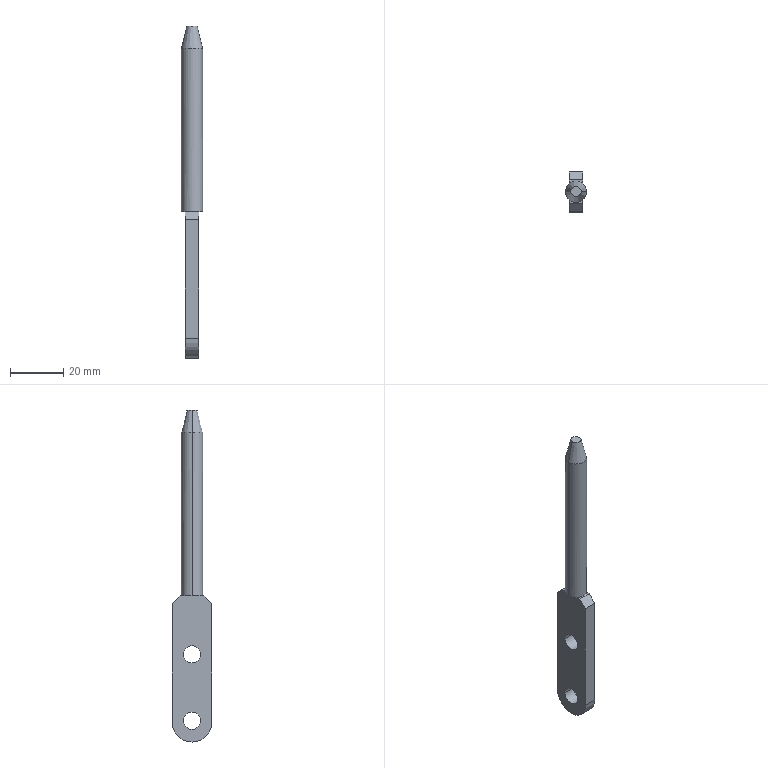Component | SolidWorks | GlassDoorAssembly-1_828LockAssembly-1_LockRod-2 | 1 solid | 21 faces | box 8 x 15 x 125 mm | volume 6966 mm3 | plane 11 | cylinder 8 | cone 2 | commonest cylinder face diameters 6.5 x4 8 x2 15 x2
STEP:
#1=CARTESIAN_POINT('',(-16.312,-19.875,-26.025));
#2=VERTEX_POINT('',#1);
#3=CARTESIAN_POINT('',(-16.312,-19.619,-26.025));
#4=VERTEX_POINT('',#3);
#5=CARTESIAN_POINT('',(-16.312,-19.747,-26.025));
#6=DIRECTION('',(-1.,-0.,-0.));
#7=DIRECTION('',(0.,1.,0.));
#8=AXIS2_PLACEMENT_3D('',#5,#6,#7);
#9=CIRCLE('',#8,0.128);
#10=EDGE_CURVE('',#2,#4,#9,.T.);
#11=ORIENTED_EDGE('',*,*,#10,.F.);
#12=CARTESIAN_POINT('',(-16.508,-19.875,-26.025));
#13=VERTEX_POINT('',#12);
#14=CARTESIAN_POINT('',(-16.312,-19.875,-26.025));
#15=DIRECTION('',(-1.,-0.,-0.));
#16=VECTOR('',#15,39.37);
#17=LINE('',#14,#16);
#18=EDGE_CURVE('',#2,#13,#17,.T.);
#19=ORIENTED_EDGE('',*,*,#18,.T.);
#20=CARTESIAN_POINT('',(-16.508,-19.619,-26.025));
#21=VERTEX_POINT('',#20);
#22=CARTESIAN_POINT('',(-16.508,-19.747,-26.025));
#23=DIRECTION('',(-1.,-0.,-0.));
#24=DIRECTION('',(0.,1.,0.));
#25=AXIS2_PLACEMENT_3D('',#22,#23,#24);
#26=CIRCLE('',#25,0.128);
#27=EDGE_CURVE('',#13,#21,#26,.T.);
#28=ORIENTED_EDGE('',*,*,#27,.T.);
#29=CARTESIAN_POINT('',(-16.312,-19.619,-26.025));
#30=DIRECTION('',(-1.,-0.,-0.));
#31=VECTOR('',#30,39.37);
#32=LINE('',#29,#31);
#33=EDGE_CURVE('',#4,#21,#32,.T.);
#34=ORIENTED_EDGE('',*,*,#33,.F.);
#35=EDGE_LOOP('',(#11,#19,#28,#34));
#36=FACE_OUTER_BOUND('',#35,.T.);
#37=CARTESIAN_POINT('',(-16.312,-19.747,-26.025));
#38=DIRECTION('',(-1.,-0.,-0.));
#39=DIRECTION('',(0.,1.,0.));
#40=AXIS2_PLACEMENT_3D('',#37,#38,#39);
#41=CYLINDRICAL_SURFACE('',#40,0.128);
#42=ADVANCED_FACE('',(#36),#41,.F.);
#43=CARTESIAN_POINT('',(-16.312,-19.875,-27.009));
#44=VERTEX_POINT('',#43);
#45=CARTESIAN_POINT('',(-16.312,-19.619,-27.009));
#46=VERTEX_POINT('',#45);
#47=CARTESIAN_POINT('',(-16.312,-19.747,-27.009));
#48=DIRECTION('',(-1.,-0.,-0.));
#49=DIRECTION('',(0.,1.,0.));
#50=AXIS2_PLACEMENT_3D('',#47,#48,#49);
#51=CIRCLE('',#50,0.128);
#52=EDGE_CURVE('',#44,#46,#51,.T.);
#53=ORIENTED_EDGE('',*,*,#52,.F.);
#54=CARTESIAN_POINT('',(-16.508,-19.875,-27.009));
#55=VERTEX_POINT('',#54);
#56=CARTESIAN_POINT('',(-16.312,-19.875,-27.009));
#57=DIRECTION('',(-1.,-0.,-0.));
#58=VECTOR('',#57,39.37);
#59=LINE('',#56,#58);
#60=EDGE_CURVE('',#44,#55,#59,.T.);
#61=ORIENTED_EDGE('',*,*,#60,.T.);
#62=CARTESIAN_POINT('',(-16.508,-19.619,-27.009));
#63=VERTEX_POINT('',#62);
#64=CARTESIAN_POINT('',(-16.508,-19.747,-27.009));
#65=DIRECTION('',(-1.,-0.,-0.));
#66=DIRECTION('',(0.,1.,0.));
#67=AXIS2_PLACEMENT_3D('',#64,#65,#66);
#68=CIRCLE('',#67,0.128);
#69=EDGE_CURVE('',#55,#63,#68,.T.);
#70=ORIENTED_EDGE('',*,*,#69,.T.);
#71=CARTESIAN_POINT('',(-16.312,-19.619,-27.009));
#72=DIRECTION('',(-1.,-0.,-0.));
#73=VECTOR('',#72,39.37);
#74=LINE('',#71,#73);
#75=EDGE_CURVE('',#46,#63,#74,.T.);
#76=ORIENTED_EDGE('',*,*,#75,.F.);
#77=EDGE_LOOP('',(#53,#61,#70,#76));
#78=FACE_OUTER_BOUND('',#77,.T.);
#79=CARTESIAN_POINT('',(-16.312,-19.747,-27.009));
#80=DIRECTION('',(-1.,-0.,-0.));
#81=DIRECTION('',(0.,1.,0.));
#82=AXIS2_PLACEMENT_3D('',#79,#80,#81);
#83=CYLINDRICAL_SURFACE('',#82,0.128);
#84=ADVANCED_FACE('',(#78),#83,.F.);
#85=CARTESIAN_POINT('',(-16.487,-19.747,-22.403));
#86=VERTEX_POINT('',#85);
#87=CARTESIAN_POINT('',(-16.333,-19.747,-22.403));
#88=VERTEX_POINT('',#87);
#89=CARTESIAN_POINT('',(-16.41,-19.747,-22.403));
#90=DIRECTION('',(0.,-0.,-1.));
#91=DIRECTION('',(-1.,0.,0.));
#92=AXIS2_PLACEMENT_3D('',#89,#90,#91);
#93=CIRCLE('',#92,0.07666);
#94=EDGE_CURVE('',#86,#88,#93,.T.);
#95=ORIENTED_EDGE('',*,*,#94,.T.);
#96=CARTESIAN_POINT('',(-16.252,-19.747,-22.734));
#97=VERTEX_POINT('',#96);
#98=CARTESIAN_POINT('',(-16.252,-19.747,-22.734));
#99=DIRECTION('',(0.2371,-0.,-0.9715));
#100=VECTOR('',#99,39.37);
#101=LINE('',#98,#100);
#102=EDGE_CURVE('',#88,#97,#101,.T.);
#103=ORIENTED_EDGE('',*,*,#102,.T.);
#104=CARTESIAN_POINT('',(-16.567,-19.747,-22.734));
#105=VERTEX_POINT('',#104);
#106=CARTESIAN_POINT('',(-16.41,-19.747,-22.734));
#107=DIRECTION('',(0.,-0.,-1.));
#108=DIRECTION('',(-1.,0.,0.));
#109=AXIS2_PLACEMENT_3D('',#106,#107,#108);
#110=CIRCLE('',#109,0.1575);
#111=EDGE_CURVE('',#105,#97,#110,.T.);
#112=ORIENTED_EDGE('',*,*,#111,.F.);
#113=CARTESIAN_POINT('',(-16.567,-19.747,-22.734));
#114=DIRECTION('',(-0.2371,-0.,-0.9715));
#115=VECTOR('',#114,39.37);
#116=LINE('',#113,#115);
#117=EDGE_CURVE('',#86,#105,#116,.T.);
#118=ORIENTED_EDGE('',*,*,#117,.F.);
#119=EDGE_LOOP('',(#95,#103,#112,#118));
#120=FACE_OUTER_BOUND('',#119,.T.);
#121=CARTESIAN_POINT('',(-16.41,-19.747,-22.734));
#122=DIRECTION('',(0.,-0.,-1.));
#123=DIRECTION('',(-1.,0.,0.));
#124=AXIS2_PLACEMENT_3D('',#121,#122,#123);
#125=CONICAL_SURFACE('',#124,0.1575,0.2394);
#126=ADVANCED_FACE('',(#120),#125,.T.);
#127=CARTESIAN_POINT('',(-16.567,-19.747,-25.159));
#128=VERTEX_POINT('',#127);
#129=CARTESIAN_POINT('',(-16.508,-19.624,-25.159));
#130=VERTEX_POINT('',#129);
#131=CARTESIAN_POINT('',(-16.41,-19.747,-25.159));
#132=DIRECTION('',(0.,-0.,-1.));
#133=DIRECTION('',(-1.,0.,0.));
#134=AXIS2_PLACEMENT_3D('',#131,#132,#133);
#135=CIRCLE('',#134,0.1575);
#136=EDGE_CURVE('',#128,#130,#135,.T.);
#137=ORIENTED_EDGE('',*,*,#136,.F.);
#138=CARTESIAN_POINT('',(-16.567,-19.747,-25.159));
#139=DIRECTION('',(-0.,0.,1.));
#140=VECTOR('',#139,39.37);
#141=LINE('',#138,#140);
#142=EDGE_CURVE('',#128,#105,#141,.T.);
#143=ORIENTED_EDGE('',*,*,#142,.T.);
#144=ORIENTED_EDGE('',*,*,#111,.T.);
#145=CARTESIAN_POINT('',(-16.252,-19.747,-25.159));
#146=VERTEX_POINT('',#145);
#147=CARTESIAN_POINT('',(-16.252,-19.747,-25.159));
#148=DIRECTION('',(-0.,0.,1.));
#149=VECTOR('',#148,39.37);
#150=LINE('',#147,#149);
#151=EDGE_CURVE('',#146,#97,#150,.T.);
#152=ORIENTED_EDGE('',*,*,#151,.F.);
#153=CARTESIAN_POINT('',(-16.312,-19.624,-25.159));
#154=VERTEX_POINT('',#153);
#155=CARTESIAN_POINT('',(-16.41,-19.747,-25.159));
#156=DIRECTION('',(0.,-0.,-1.));
#157=DIRECTION('',(-1.,0.,0.));
#158=AXIS2_PLACEMENT_3D('',#155,#156,#157);
#159=CIRCLE('',#158,0.1575);
#160=EDGE_CURVE('',#154,#146,#159,.T.);
#161=ORIENTED_EDGE('',*,*,#160,.F.);
#162=CARTESIAN_POINT('',(-16.41,-19.747,-25.159));
#163=DIRECTION('',(0.,-0.,-1.));
#164=DIRECTION('',(-1.,0.,0.));
#165=AXIS2_PLACEMENT_3D('',#162,#163,#164);
#166=CIRCLE('',#165,0.1575);
#167=EDGE_CURVE('',#130,#154,#166,.T.);
#168=ORIENTED_EDGE('',*,*,#167,.F.);
#169=EDGE_LOOP('',(#137,#143,#144,#152,#161,#168));
#170=FACE_OUTER_BOUND('',#169,.T.);
#171=CARTESIAN_POINT('',(-16.41,-19.747,-25.159));
#172=DIRECTION('',(-0.,0.,1.));
#173=DIRECTION('',(1.,0.,0.));
#174=AXIS2_PLACEMENT_3D('',#171,#172,#173);
#175=CYLINDRICAL_SURFACE('',#174,0.1575);
#176=ADVANCED_FACE('',(#170),#175,.T.);
#177=CARTESIAN_POINT('',(-16.508,-19.87,-25.159));
#178=VERTEX_POINT('',#177);
#179=CARTESIAN_POINT('',(-16.508,-19.452,-25.159));
#180=DIRECTION('',(-0.,1.,-0.));
#181=VECTOR('',#180,39.37);
#182=LINE('',#179,#181);
#183=EDGE_CURVE('',#178,#130,#182,.T.);
#184=ORIENTED_EDGE('',*,*,#183,.F.);
#185=CARTESIAN_POINT('',(-16.41,-19.747,-25.159));
#186=DIRECTION('',(0.,-0.,-1.));
#187=DIRECTION('',(-1.,0.,0.));
#188=AXIS2_PLACEMENT_3D('',#185,#186,#187);
#189=CIRCLE('',#188,0.1575);
#190=EDGE_CURVE('',#178,#128,#189,.T.);
#191=ORIENTED_EDGE('',*,*,#190,.T.);
#192=ORIENTED_EDGE('',*,*,#136,.T.);
#193=EDGE_LOOP('',(#184,#191,#192));
#194=FACE_OUTER_BOUND('',#193,.T.);
#195=CARTESIAN_POINT('',(-16.41,-19.747,-25.159));
#196=DIRECTION('',(0.,-0.,-1.));
#197=DIRECTION('',(-1.,-0.,-0.));
#198=AXIS2_PLACEMENT_3D('',#195,#196,#197);
#199=PLANE('',#198);
#200=ADVANCED_FACE('',(#194),#199,.T.);
#201=ORIENTED_EDGE('',*,*,#142,.F.);
#202=ORIENTED_EDGE('',*,*,#190,.F.);
#203=CARTESIAN_POINT('',(-16.312,-19.87,-25.159));
#204=VERTEX_POINT('',#203);
#205=CARTESIAN_POINT('',(-16.41,-19.747,-25.159));
#206=DIRECTION('',(0.,-0.,-1.));
#207=DIRECTION('',(-1.,0.,0.));
#208=AXIS2_PLACEMENT_3D('',#205,#206,#207);
#209=CIRCLE('',#208,0.1575);
#210=EDGE_CURVE('',#204,#178,#209,.T.);
#211=ORIENTED_EDGE('',*,*,#210,.F.);
#212=CARTESIAN_POINT('',(-16.41,-19.747,-25.159));
#213=DIRECTION('',(0.,-0.,-1.));
#214=DIRECTION('',(-1.,0.,0.));
#215=AXIS2_PLACEMENT_3D('',#212,#213,#214);
#216=CIRCLE('',#215,0.1575);
#217=EDGE_CURVE('',#146,#204,#216,.T.);
#218=ORIENTED_EDGE('',*,*,#217,.F.);
#219=ORIENTED_EDGE('',*,*,#151,.T.);
#220=CARTESIAN_POINT('',(-16.41,-19.747,-22.734));
#221=DIRECTION('',(0.,-0.,-1.));
#222=DIRECTION('',(-1.,0.,0.));
#223=AXIS2_PLACEMENT_3D('',#220,#221,#222);
#224=CIRCLE('',#223,0.1575);
#225=EDGE_CURVE('',#97,#105,#224,.T.);
#226=ORIENTED_EDGE('',*,*,#225,.T.);
#227=EDGE_LOOP('',(#201,#202,#211,#218,#219,#226));
#228=FACE_OUTER_BOUND('',#227,.T.);
#229=CARTESIAN_POINT('',(-16.41,-19.747,-25.159));
#230=DIRECTION('',(-0.,0.,1.));
#231=DIRECTION('',(1.,0.,0.));
#232=AXIS2_PLACEMENT_3D('',#229,#230,#231);
#233=CYLINDRICAL_SURFACE('',#232,0.1575);
#234=ADVANCED_FACE('',(#228),#233,.T.);
#235=CARTESIAN_POINT('',(-16.312,-19.452,-25.159));
#236=DIRECTION('',(0.,-1.,0.));
#237=VECTOR('',#236,39.37);
#238=LINE('',#235,#237);
#239=EDGE_CURVE('',#154,#204,#238,.T.);
#240=ORIENTED_EDGE('',*,*,#239,.F.);
#241=ORIENTED_EDGE('',*,*,#160,.T.);
#242=ORIENTED_EDGE('',*,*,#217,.T.);
#243=EDGE_LOOP('',(#240,#241,#242));
#244=FACE_OUTER_BOUND('',#243,.T.);
#245=CARTESIAN_POINT('',(-16.41,-19.747,-25.159));
#246=DIRECTION('',(0.,-0.,-1.));
#247=DIRECTION('',(-1.,-0.,-0.));
#248=AXIS2_PLACEMENT_3D('',#245,#246,#247);
#249=PLANE('',#248);
#250=ADVANCED_FACE('',(#244),#249,.T.);
#251=ORIENTED_EDGE('',*,*,#102,.F.);
#252=CARTESIAN_POINT('',(-16.41,-19.747,-22.403));
#253=DIRECTION('',(0.,-0.,-1.));
#254=DIRECTION('',(-1.,0.,0.));
#255=AXIS2_PLACEMENT_3D('',#252,#253,#254);
#256=CIRCLE('',#255,0.07666);
#257=EDGE_CURVE('',#88,#86,#256,.T.);
#258=ORIENTED_EDGE('',*,*,#257,.T.);
#259=ORIENTED_EDGE('',*,*,#117,.T.);
#260=ORIENTED_EDGE('',*,*,#225,.F.);
#261=EDGE_LOOP('',(#251,#258,#259,#260));
#262=FACE_OUTER_BOUND('',#261,.T.);
#263=CARTESIAN_POINT('',(-16.41,-19.747,-22.734));
#264=DIRECTION('',(0.,-0.,-1.));
#265=DIRECTION('',(-1.,0.,0.));
#266=AXIS2_PLACEMENT_3D('',#263,#264,#265);
#267=CONICAL_SURFACE('',#266,0.1575,0.2394);
#268=ADVANCED_FACE('',(#262),#267,.T.);
#269=ORIENTED_EDGE('',*,*,#94,.F.);
#270=ORIENTED_EDGE('',*,*,#257,.F.);
#271=EDGE_LOOP('',(#269,#270));
#272=FACE_OUTER_BOUND('',#271,.T.);
#273=CARTESIAN_POINT('',(-16.41,-19.747,-22.403));
#274=DIRECTION('',(0.,-0.,-1.));
#275=DIRECTION('',(-1.,-0.,-0.));
#276=AXIS2_PLACEMENT_3D('',#273,#274,#275);
#277=PLANE('',#276);
#278=ADVANCED_FACE('',(#272),#277,.F.);
#279=CARTESIAN_POINT('',(-16.312,-19.57,-25.159));
#280=VERTEX_POINT('',#279);
#281=CARTESIAN_POINT('',(-16.312,-19.452,-25.159));
#282=DIRECTION('',(0.,-1.,0.));
#283=VECTOR('',#282,39.37);
#284=LINE('',#281,#283);
#285=EDGE_CURVE('',#280,#154,#284,.T.);
#286=ORIENTED_EDGE('',*,*,#285,.F.);
#287=CARTESIAN_POINT('',(-16.508,-19.57,-25.159));
#288=VERTEX_POINT('',#287);
#289=CARTESIAN_POINT('',(-16.508,-19.57,-25.159));
#290=DIRECTION('',(-1.,-0.,-0.));
#291=VECTOR('',#290,39.37);
#292=LINE('',#289,#291);
#293=EDGE_CURVE('',#280,#288,#292,.T.);
#294=ORIENTED_EDGE('',*,*,#293,.T.);
#295=CARTESIAN_POINT('',(-16.508,-19.452,-25.159));
#296=DIRECTION('',(-0.,1.,-0.));
#297=VECTOR('',#296,39.37);
#298=LINE('',#295,#297);
#299=EDGE_CURVE('',#130,#288,#298,.T.);
#300=ORIENTED_EDGE('',*,*,#299,.F.);
#301=ORIENTED_EDGE('',*,*,#167,.T.);
#302=EDGE_LOOP('',(#286,#294,#300,#301));
#303=FACE_OUTER_BOUND('',#302,.T.);
#304=CARTESIAN_POINT('',(-16.508,-20.042,-25.159));
#305=DIRECTION('',(0.,-0.,-1.));
#306=DIRECTION('',(-1.,-0.,-0.));
#307=AXIS2_PLACEMENT_3D('',#304,#305,#306);
#308=PLANE('',#307);
#309=ADVANCED_FACE('',(#303),#308,.F.);
#310=CARTESIAN_POINT('',(-16.508,-19.924,-25.159));
#311=VERTEX_POINT('',#310);
#312=CARTESIAN_POINT('',(-16.508,-19.452,-25.159));
#313=DIRECTION('',(-0.,1.,-0.));
#314=VECTOR('',#313,39.37);
#315=LINE('',#312,#314);
#316=EDGE_CURVE('',#311,#178,#315,.T.);
#317=ORIENTED_EDGE('',*,*,#316,.F.);
#318=CARTESIAN_POINT('',(-16.312,-19.924,-25.159));
#319=VERTEX_POINT('',#318);
#320=CARTESIAN_POINT('',(-16.508,-19.924,-25.159));
#321=DIRECTION('',(1.,0.,0.));
#322=VECTOR('',#321,39.37);
#323=LINE('',#320,#322);
#324=EDGE_CURVE('',#311,#319,#323,.T.);
#325=ORIENTED_EDGE('',*,*,#324,.T.);
#326=CARTESIAN_POINT('',(-16.312,-19.452,-25.159));
#327=DIRECTION('',(0.,-1.,0.));
#328=VECTOR('',#327,39.37);
#329=LINE('',#326,#328);
#330=EDGE_CURVE('',#204,#319,#329,.T.);
#331=ORIENTED_EDGE('',*,*,#330,.F.);
#332=ORIENTED_EDGE('',*,*,#210,.T.);
#333=EDGE_LOOP('',(#317,#325,#331,#332));
#334=FACE_OUTER_BOUND('',#333,.T.);
#335=CARTESIAN_POINT('',(-16.508,-20.042,-25.159));
#336=DIRECTION('',(0.,-0.,-1.));
#337=DIRECTION('',(-1.,-0.,-0.));
#338=AXIS2_PLACEMENT_3D('',#335,#336,#337);
#339=PLANE('',#338);
#340=ADVANCED_FACE('',(#334),#339,.F.);
#341=CARTESIAN_POINT('',(-16.508,-19.747,-26.025));
#342=DIRECTION('',(-1.,-0.,-0.));
#343=DIRECTION('',(0.,1.,0.));
#344=AXIS2_PLACEMENT_3D('',#341,#342,#343);
#345=CIRCLE('',#344,0.128);
#346=EDGE_CURVE('',#21,#13,#345,.T.);
#347=ORIENTED_EDGE('',*,*,#346,.F.);
#348=ORIENTED_EDGE('',*,*,#27,.F.);
#349=EDGE_LOOP('',(#347,#348));
#350=FACE_BOUND('',#349,.T.);
#351=CARTESIAN_POINT('',(-16.508,-19.747,-27.009));
#352=DIRECTION('',(-1.,-0.,-0.));
#353=DIRECTION('',(0.,1.,0.));
#354=AXIS2_PLACEMENT_3D('',#351,#352,#353);
#355=CIRCLE('',#354,0.128);
#356=EDGE_CURVE('',#63,#55,#355,.T.);
#357=ORIENTED_EDGE('',*,*,#356,.F.);
#358=ORIENTED_EDGE('',*,*,#69,.F.);
#359=EDGE_LOOP('',(#357,#358));
#360=FACE_BOUND('',#359,.T.);
#361=CARTESIAN_POINT('',(-16.508,-19.452,-27.029));
#362=VERTEX_POINT('',#361);
#363=CARTESIAN_POINT('',(-16.508,-19.747,-27.324));
#364=VERTEX_POINT('',#363);
#365=CARTESIAN_POINT('',(-16.508,-19.747,-27.029));
#366=DIRECTION('',(-1.,-0.,-0.));
#367=DIRECTION('',(0.,-1.,0.));
#368=AXIS2_PLACEMENT_3D('',#365,#366,#367);
#369=CIRCLE('',#368,0.2953);
#370=EDGE_CURVE('',#362,#364,#369,.T.);
#371=ORIENTED_EDGE('',*,*,#370,.T.);
#372=CARTESIAN_POINT('',(-16.508,-20.042,-27.029));
#373=VERTEX_POINT('',#372);
#374=CARTESIAN_POINT('',(-16.508,-19.747,-27.029));
#375=DIRECTION('',(-1.,-0.,-0.));
#376=DIRECTION('',(0.,-1.,0.));
#377=AXIS2_PLACEMENT_3D('',#374,#375,#376);
#378=CIRCLE('',#377,0.2953);
#379=EDGE_CURVE('',#364,#373,#378,.T.);
#380=ORIENTED_EDGE('',*,*,#379,.T.);
#381=CARTESIAN_POINT('',(-16.508,-20.042,-25.277));
#382=VERTEX_POINT('',#381);
#383=CARTESIAN_POINT('',(-16.508,-20.042,-27.324));
#384=DIRECTION('',(-0.,0.,1.));
#385=VECTOR('',#384,39.37);
#386=LINE('',#383,#385);
#387=EDGE_CURVE('',#373,#382,#386,.T.);
#388=ORIENTED_EDGE('',*,*,#387,.T.);
#389=CARTESIAN_POINT('',(-16.508,-20.042,-25.277));
#390=DIRECTION('',(-0.,0.7071,0.7071));
#391=VECTOR('',#390,39.37);
#392=LINE('',#389,#391);
#393=EDGE_CURVE('',#382,#311,#392,.T.);
#394=ORIENTED_EDGE('',*,*,#393,.T.);
#395=ORIENTED_EDGE('',*,*,#316,.T.);
#396=ORIENTED_EDGE('',*,*,#183,.T.);
#397=ORIENTED_EDGE('',*,*,#299,.T.);
#398=CARTESIAN_POINT('',(-16.508,-19.452,-25.277));
#399=VERTEX_POINT('',#398);
#400=CARTESIAN_POINT('',(-16.508,-19.452,-25.277));
#401=DIRECTION('',(0.,0.7071,-0.7071));
#402=VECTOR('',#401,39.37);
#403=LINE('',#400,#402);
#404=EDGE_CURVE('',#288,#399,#403,.T.);
#405=ORIENTED_EDGE('',*,*,#404,.T.);
#406=CARTESIAN_POINT('',(-16.508,-19.452,-27.324));
#407=DIRECTION('',(-0.,0.,1.));
#408=VECTOR('',#407,39.37);
#409=LINE('',#406,#408);
#410=EDGE_CURVE('',#362,#399,#409,.T.);
#411=ORIENTED_EDGE('',*,*,#410,.F.);
#412=EDGE_LOOP('',(#371,#380,#388,#394,#395,#396,#397,#405,#411));
#413=FACE_OUTER_BOUND('',#412,.T.);
#414=CARTESIAN_POINT('',(-16.508,-19.452,-27.324));
#415=DIRECTION('',(1.,0.,0.));
#416=DIRECTION('',(0.,-1.,0.));
#417=AXIS2_PLACEMENT_3D('',#414,#415,#416);
#418=PLANE('',#417);
#419=ADVANCED_FACE('',(#350,#360,#413),#418,.F.);
#420=CARTESIAN_POINT('',(-16.312,-19.452,-27.029));
#421=VERTEX_POINT('',#420);
#422=CARTESIAN_POINT('',(-16.312,-19.452,-25.277));
#423=VERTEX_POINT('',#422);
#424=CARTESIAN_POINT('',(-16.312,-19.452,-27.324));
#425=DIRECTION('',(-0.,0.,1.));
#426=VECTOR('',#425,39.37);
#427=LINE('',#424,#426);
#428=EDGE_CURVE('',#421,#423,#427,.T.);
#429=ORIENTED_EDGE('',*,*,#428,.F.);
#430=CARTESIAN_POINT('',(-16.508,-19.452,-27.029));
#431=DIRECTION('',(-1.,-0.,-0.));
#432=VECTOR('',#431,39.37);
#433=LINE('',#430,#432);
#434=EDGE_CURVE('',#421,#362,#433,.T.);
#435=ORIENTED_EDGE('',*,*,#434,.T.);
#436=ORIENTED_EDGE('',*,*,#410,.T.);
#437=CARTESIAN_POINT('',(-16.312,-19.452,-25.277));
#438=DIRECTION('',(1.,0.,0.));
#439=VECTOR('',#438,39.37);
#440=LINE('',#437,#439);
#441=EDGE_CURVE('',#399,#423,#440,.T.);
#442=ORIENTED_EDGE('',*,*,#441,.T.);
#443=EDGE_LOOP('',(#429,#435,#436,#442));
#444=FACE_OUTER_BOUND('',#443,.T.);
#445=CARTESIAN_POINT('',(-16.312,-19.452,-27.324));
#446=DIRECTION('',(0.,-1.,0.));
#447=DIRECTION('',(-0.,0.,1.));
#448=AXIS2_PLACEMENT_3D('',#445,#446,#447);
#449=PLANE('',#448);
#450=ADVANCED_FACE('',(#444),#449,.F.);
#451=CARTESIAN_POINT('',(-16.312,-19.747,-26.025));
#452=DIRECTION('',(-1.,-0.,-0.));
#453=DIRECTION('',(0.,1.,0.));
#454=AXIS2_PLACEMENT_3D('',#451,#452,#453);
#455=CIRCLE('',#454,0.128);
#456=EDGE_CURVE('',#4,#2,#455,.T.);
#457=ORIENTED_EDGE('',*,*,#456,.T.);
#458=ORIENTED_EDGE('',*,*,#10,.T.);
#459=EDGE_LOOP('',(#457,#458));
#460=FACE_BOUND('',#459,.T.);
#461=CARTESIAN_POINT('',(-16.312,-19.747,-27.009));
#462=DIRECTION('',(-1.,-0.,-0.));
#463=DIRECTION('',(0.,1.,0.));
#464=AXIS2_PLACEMENT_3D('',#461,#462,#463);
#465=CIRCLE('',#464,0.128);
#466=EDGE_CURVE('',#46,#44,#465,.T.);
#467=ORIENTED_EDGE('',*,*,#466,.T.);
#468=ORIENTED_EDGE('',*,*,#52,.T.);
#469=EDGE_LOOP('',(#467,#468));
#470=FACE_BOUND('',#469,.T.);
#471=CARTESIAN_POINT('',(-16.312,-20.042,-27.029));
#472=VERTEX_POINT('',#471);
#473=CARTESIAN_POINT('',(-16.312,-20.042,-25.277));
#474=VERTEX_POINT('',#473);
#475=CARTESIAN_POINT('',(-16.312,-20.042,-27.324));
#476=DIRECTION('',(-0.,0.,1.));
#477=VECTOR('',#476,39.37);
#478=LINE('',#475,#477);
#479=EDGE_CURVE('',#472,#474,#478,.T.);
#480=ORIENTED_EDGE('',*,*,#479,.F.);
#481=CARTESIAN_POINT('',(-16.312,-19.747,-27.324));
#482=VERTEX_POINT('',#481);
#483=CARTESIAN_POINT('',(-16.312,-19.747,-27.029));
#484=DIRECTION('',(1.,0.,0.));
#485=DIRECTION('',(0.,1.,0.));
#486=AXIS2_PLACEMENT_3D('',#483,#484,#485);
#487=CIRCLE('',#486,0.2953);
#488=EDGE_CURVE('',#472,#482,#487,.T.);
#489=ORIENTED_EDGE('',*,*,#488,.T.);
#490=CARTESIAN_POINT('',(-16.312,-19.747,-27.029));
#491=DIRECTION('',(1.,0.,0.));
#492=DIRECTION('',(0.,1.,0.));
#493=AXIS2_PLACEMENT_3D('',#490,#491,#492);
#494=CIRCLE('',#493,0.2953);
#495=EDGE_CURVE('',#482,#421,#494,.T.);
#496=ORIENTED_EDGE('',*,*,#495,.T.);
#497=ORIENTED_EDGE('',*,*,#428,.T.);
#498=CARTESIAN_POINT('',(-16.312,-19.452,-25.277));
#499=DIRECTION('',(-0.,-0.7071,0.7071));
#500=VECTOR('',#499,39.37);
#501=LINE('',#498,#500);
#502=EDGE_CURVE('',#423,#280,#501,.T.);
#503=ORIENTED_EDGE('',*,*,#502,.T.);
#504=ORIENTED_EDGE('',*,*,#285,.T.);
#505=ORIENTED_EDGE('',*,*,#239,.T.);
#506=ORIENTED_EDGE('',*,*,#330,.T.);
#507=CARTESIAN_POINT('',(-16.312,-20.042,-25.277));
#508=DIRECTION('',(0.,-0.7071,-0.7071));
#509=VECTOR('',#508,39.37);
#510=LINE('',#507,#509);
#511=EDGE_CURVE('',#319,#474,#510,.T.);
#512=ORIENTED_EDGE('',*,*,#511,.T.);
#513=EDGE_LOOP('',(#480,#489,#496,#497,#503,#504,#505,#506,#512));
#514=FACE_OUTER_BOUND('',#513,.T.);
#515=CARTESIAN_POINT('',(-16.312,-19.452,-27.324));
#516=DIRECTION('',(-1.,-0.,-0.));
#517=DIRECTION('',(-0.,1.,-0.));
#518=AXIS2_PLACEMENT_3D('',#515,#516,#517);
#519=PLANE('',#518);
#520=ADVANCED_FACE('',(#460,#470,#514),#519,.F.);
#521=ORIENTED_EDGE('',*,*,#387,.F.);
#522=CARTESIAN_POINT('',(-16.312,-20.042,-27.029));
#523=DIRECTION('',(1.,0.,0.));
#524=VECTOR('',#523,39.37);
#525=LINE('',#522,#524);
#526=EDGE_CURVE('',#373,#472,#525,.T.);
#527=ORIENTED_EDGE('',*,*,#526,.T.);
#528=ORIENTED_EDGE('',*,*,#479,.T.);
#529=CARTESIAN_POINT('',(-16.312,-20.042,-25.277));
#530=DIRECTION('',(-1.,-0.,-0.));
#531=VECTOR('',#530,39.37);
#532=LINE('',#529,#531);
#533=EDGE_CURVE('',#474,#382,#532,.T.);
#534=ORIENTED_EDGE('',*,*,#533,.T.);
#535=EDGE_LOOP('',(#521,#527,#528,#534));
#536=FACE_OUTER_BOUND('',#535,.T.);
#537=CARTESIAN_POINT('',(-16.312,-20.042,-27.324));
#538=DIRECTION('',(-0.,1.,-0.));
#539=DIRECTION('',(0.,-0.,-1.));
#540=AXIS2_PLACEMENT_3D('',#537,#538,#539);
#541=PLANE('',#540);
#542=ADVANCED_FACE('',(#536),#541,.F.);
#543=ORIENTED_EDGE('',*,*,#511,.F.);
#544=ORIENTED_EDGE('',*,*,#324,.F.);
#545=ORIENTED_EDGE('',*,*,#393,.F.);
#546=ORIENTED_EDGE('',*,*,#533,.F.);
#547=EDGE_LOOP('',(#543,#544,#545,#546));
#548=FACE_OUTER_BOUND('',#547,.T.);
#549=CARTESIAN_POINT('',(-16.312,-20.042,-25.277));
#550=DIRECTION('',(0.,0.7071,-0.7071));
#551=DIRECTION('',(0.,-0.7071,-0.7071));
#552=AXIS2_PLACEMENT_3D('',#549,#550,#551);
#553=PLANE('',#552);
#554=ADVANCED_FACE('',(#548),#553,.F.);
#555=ORIENTED_EDGE('',*,*,#404,.F.);
#556=ORIENTED_EDGE('',*,*,#293,.F.);
#557=ORIENTED_EDGE('',*,*,#502,.F.);
#558=ORIENTED_EDGE('',*,*,#441,.F.);
#559=EDGE_LOOP('',(#555,#556,#557,#558));
#560=FACE_OUTER_BOUND('',#559,.T.);
#561=CARTESIAN_POINT('',(-16.312,-19.452,-25.277));
#562=DIRECTION('',(0.,-0.7071,-0.7071));
#563=DIRECTION('',(-0.,-0.7071,0.7071));
#564=AXIS2_PLACEMENT_3D('',#561,#562,#563);
#565=PLANE('',#564);
#566=ADVANCED_FACE('',(#560),#565,.F.);
#567=ORIENTED_EDGE('',*,*,#60,.F.);
#568=ORIENTED_EDGE('',*,*,#466,.F.);
#569=ORIENTED_EDGE('',*,*,#75,.T.);
#570=ORIENTED_EDGE('',*,*,#356,.T.);
#571=EDGE_LOOP('',(#567,#568,#569,#570));
#572=FACE_OUTER_BOUND('',#571,.T.);
#573=CARTESIAN_POINT('',(-16.312,-19.747,-27.009));
#574=DIRECTION('',(-1.,-0.,-0.));
#575=DIRECTION('',(0.,1.,0.));
#576=AXIS2_PLACEMENT_3D('',#573,#574,#575);
#577=CYLINDRICAL_SURFACE('',#576,0.128);
#578=ADVANCED_FACE('',(#572),#577,.F.);
#579=ORIENTED_EDGE('',*,*,#18,.F.);
#580=ORIENTED_EDGE('',*,*,#456,.F.);
#581=ORIENTED_EDGE('',*,*,#33,.T.);
#582=ORIENTED_EDGE('',*,*,#346,.T.);
#583=EDGE_LOOP('',(#579,#580,#581,#582));
#584=FACE_OUTER_BOUND('',#583,.T.);
#585=CARTESIAN_POINT('',(-16.312,-19.747,-26.025));
#586=DIRECTION('',(-1.,-0.,-0.));
#587=DIRECTION('',(0.,1.,0.));
#588=AXIS2_PLACEMENT_3D('',#585,#586,#587);
#589=CYLINDRICAL_SURFACE('',#588,0.128);
#590=ADVANCED_FACE('',(#584),#589,.F.);
#591=ORIENTED_EDGE('',*,*,#434,.F.);
#592=ORIENTED_EDGE('',*,*,#495,.F.);
#593=CARTESIAN_POINT('',(-16.312,-19.747,-27.324));
#594=DIRECTION('',(1.,0.,0.));
#595=VECTOR('',#594,39.37);
#596=LINE('',#593,#595);
#597=EDGE_CURVE('',#364,#482,#596,.T.);
#598=ORIENTED_EDGE('',*,*,#597,.F.);
#599=ORIENTED_EDGE('',*,*,#370,.F.);
#600=EDGE_LOOP('',(#591,#592,#598,#599));
#601=FACE_OUTER_BOUND('',#600,.T.);
#602=CARTESIAN_POINT('',(-16.508,-19.747,-27.029));
#603=DIRECTION('',(-1.,-0.,-0.));
#604=DIRECTION('',(0.,0.,1.));
#605=AXIS2_PLACEMENT_3D('',#602,#603,#604);
#606=CYLINDRICAL_SURFACE('',#605,0.2953);
#607=ADVANCED_FACE('',(#601),#606,.T.);
#608=ORIENTED_EDGE('',*,*,#488,.F.);
#609=ORIENTED_EDGE('',*,*,#526,.F.);
#610=ORIENTED_EDGE('',*,*,#379,.F.);
#611=ORIENTED_EDGE('',*,*,#597,.T.);
#612=EDGE_LOOP('',(#608,#609,#610,#611));
#613=FACE_OUTER_BOUND('',#612,.T.);
#614=CARTESIAN_POINT('',(-16.508,-19.747,-27.029));
#615=DIRECTION('',(1.,0.,0.));
#616=DIRECTION('',(0.,0.,-1.));
#617=AXIS2_PLACEMENT_3D('',#614,#615,#616);
#618=CYLINDRICAL_SURFACE('',#617,0.2953);
#619=ADVANCED_FACE('',(#613),#618,.T.);
#620=CLOSED_SHELL('',(#42,#84,#126,#176,#200,#234,#250,#268,#278,#309,#340,#419,#450,#520,#542,#554,#566,#578,#590,#607,#619));
#621=MANIFOLD_SOLID_BREP('',#620);
#622=CARTESIAN_POINT('',(0.,0.,0.));
#623=DIRECTION('',(0.,0.,1.));
#624=DIRECTION('',(1.,0.,0.));
#625=AXIS2_PLACEMENT_3D('',#622,#623,#624);
#626=(LENGTH_UNIT()NAMED_UNIT(*)SI_UNIT($,.METRE.));
#627=LENGTH_MEASURE_WITH_UNIT(LENGTH_MEASURE(0.0254),#626);
#628=DIMENSIONAL_EXPONENTS(1.,0.,0.,0.,0.,0.,0.);
#629=(CONVERSION_BASED_UNIT('',#627)LENGTH_UNIT()NAMED_UNIT(#628));
#630=UNCERTAINTY_MEASURE_WITH_UNIT(LENGTH_MEASURE(0.00001),#629,'','');
#631=(NAMED_UNIT(*)PLANE_ANGLE_UNIT()SI_UNIT($,.RADIAN.));
#632=(NAMED_UNIT(*)SI_UNIT($,.STERADIAN.)SOLID_ANGLE_UNIT());
#633=(GEOMETRIC_REPRESENTATION_CONTEXT(3)GLOBAL_UNCERTAINTY_ASSIGNED_CONTEXT((#630))GLOBAL_UNIT_ASSIGNED_CONTEXT((#629,#631,#632))REPRESENTATION_CONTEXT('',''));
#634=ADVANCED_BREP_SHAPE_REPRESENTATION('',(#621,#625),#633);
#635=COLOUR_RGB('',0.7922,0.8196,0.9333);
#636=FILL_AREA_STYLE_COLOUR('',#635);
#637=FILL_AREA_STYLE('',(#636));
#638=SURFACE_STYLE_FILL_AREA(#637);
#639=SURFACE_SIDE_STYLE('',(#638));
#640=SURFACE_STYLE_USAGE(.BOTH.,#639);
#641=PRESENTATION_STYLE_ASSIGNMENT((#640));
#642=STYLED_ITEM('',(#641),#621);
#643=PRESENTATION_LAYER_ASSIGNMENT('','',(#642));
#644=(LENGTH_UNIT()NAMED_UNIT(*)SI_UNIT($,.METRE.));
#645=LENGTH_MEASURE_WITH_UNIT(LENGTH_MEASURE(0.0254),#644);
#646=DIMENSIONAL_EXPONENTS(1.,0.,0.,0.,0.,0.,0.);
#647=(CONVERSION_BASED_UNIT('',#645)LENGTH_UNIT()NAMED_UNIT(#646));
#648=UNCERTAINTY_MEASURE_WITH_UNIT(LENGTH_MEASURE(0.00001),#647,'','');
#649=(NAMED_UNIT(*)PLANE_ANGLE_UNIT()SI_UNIT($,.RADIAN.));
#650=(NAMED_UNIT(*)SI_UNIT($,.STERADIAN.)SOLID_ANGLE_UNIT());
#651=(GEOMETRIC_REPRESENTATION_CONTEXT(3)GLOBAL_UNCERTAINTY_ASSIGNED_CONTEXT((#648))GLOBAL_UNIT_ASSIGNED_CONTEXT((#647,#649,#650))REPRESENTATION_CONTEXT('',''));
#652=MECHANICAL_DESIGN_GEOMETRIC_PRESENTATION_REPRESENTATION('',(#642),#651);